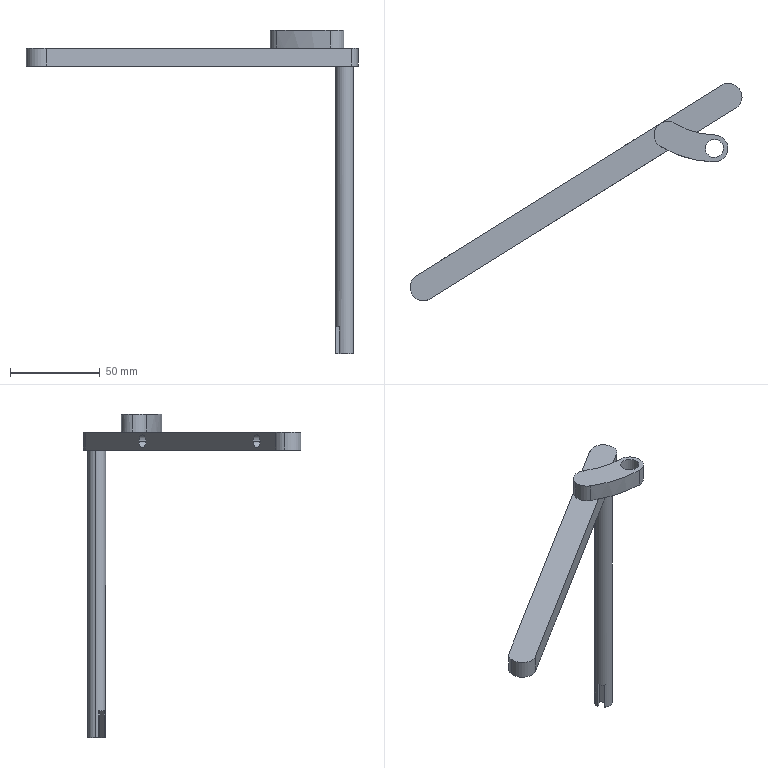Component | SolidWorks | DRocker(Left)-2 | 1 solid | 30 faces | box 184.66 x 120.91 x 180 mm | volume 48377 mm3 | cylinder 16 | plane 14 | commonest cylinder face diameters 15 x6 7 x4 10 x4 120 x1 90 x1
STEP:
#1=CARTESIAN_POINT('',(-10.505,0.6099,4.81));
#2=VERTEX_POINT('',#1);
#3=CARTESIAN_POINT('',(-10.738,0.464,4.81));
#4=VERTEX_POINT('',#3);
#5=CARTESIAN_POINT('',(-10.621,0.537,4.81));
#6=DIRECTION('',(-0.5295,0.8483,0.));
#7=DIRECTION('',(-0.8483,-0.5295,0.));
#8=AXIS2_PLACEMENT_3D('',#5,#6,#7);
#9=CIRCLE('',#8,0.1378);
#10=EDGE_CURVE('',#2,#4,#9,.T.);
#11=ORIENTED_EDGE('',*,*,#10,.F.);
#12=CARTESIAN_POINT('',(-10.713,0.9439,4.81));
#13=VERTEX_POINT('',#12);
#14=CARTESIAN_POINT('',(-10.505,0.6099,4.81));
#15=DIRECTION('',(-0.5295,0.8483,0.));
#16=VECTOR('',#15,39.37);
#17=LINE('',#14,#16);
#18=EDGE_CURVE('',#2,#13,#17,.T.);
#19=ORIENTED_EDGE('',*,*,#18,.T.);
#20=CARTESIAN_POINT('',(-10.947,0.798,4.81));
#21=VERTEX_POINT('',#20);
#22=CARTESIAN_POINT('',(-10.83,0.8709,4.81));
#23=DIRECTION('',(-0.5295,0.8483,0.));
#24=DIRECTION('',(-0.8483,-0.5295,0.));
#25=AXIS2_PLACEMENT_3D('',#22,#23,#24);
#26=CIRCLE('',#25,0.1378);
#27=EDGE_CURVE('',#13,#21,#26,.T.);
#28=ORIENTED_EDGE('',*,*,#27,.T.);
#29=CARTESIAN_POINT('',(-10.738,0.464,4.81));
#30=DIRECTION('',(-0.5295,0.8483,0.));
#31=VECTOR('',#30,39.37);
#32=LINE('',#29,#31);
#33=EDGE_CURVE('',#4,#21,#32,.T.);
#34=ORIENTED_EDGE('',*,*,#33,.F.);
#35=EDGE_LOOP('',(#11,#19,#28,#34));
#36=FACE_OUTER_BOUND('',#35,.T.);
#37=CARTESIAN_POINT('',(-10.621,0.537,4.81));
#38=DIRECTION('',(-0.5295,0.8483,0.));
#39=DIRECTION('',(-0.8483,-0.5295,0.));
#40=AXIS2_PLACEMENT_3D('',#37,#38,#39);
#41=CYLINDRICAL_SURFACE('',#40,0.1378);
#42=ADVANCED_FACE('',(#36),#41,.F.);
#43=CARTESIAN_POINT('',(-14.512,-1.892,4.81));
#44=VERTEX_POINT('',#43);
#45=CARTESIAN_POINT('',(-14.746,-2.038,4.81));
#46=VERTEX_POINT('',#45);
#47=CARTESIAN_POINT('',(-14.629,-1.965,4.81));
#48=DIRECTION('',(-0.5295,0.8483,0.));
#49=DIRECTION('',(-0.8483,-0.5295,0.));
#50=AXIS2_PLACEMENT_3D('',#47,#48,#49);
#51=CIRCLE('',#50,0.1378);
#52=EDGE_CURVE('',#44,#46,#51,.T.);
#53=ORIENTED_EDGE('',*,*,#52,.F.);
#54=CARTESIAN_POINT('',(-14.721,-1.558,4.81));
#55=VERTEX_POINT('',#54);
#56=CARTESIAN_POINT('',(-14.512,-1.892,4.81));
#57=DIRECTION('',(-0.5295,0.8483,0.));
#58=VECTOR('',#57,39.37);
#59=LINE('',#56,#58);
#60=EDGE_CURVE('',#44,#55,#59,.T.);
#61=ORIENTED_EDGE('',*,*,#60,.T.);
#62=CARTESIAN_POINT('',(-14.954,-1.704,4.81));
#63=VERTEX_POINT('',#62);
#64=CARTESIAN_POINT('',(-14.838,-1.631,4.81));
#65=DIRECTION('',(-0.5295,0.8483,0.));
#66=DIRECTION('',(-0.8483,-0.5295,0.));
#67=AXIS2_PLACEMENT_3D('',#64,#65,#66);
#68=CIRCLE('',#67,0.1378);
#69=EDGE_CURVE('',#55,#63,#68,.T.);
#70=ORIENTED_EDGE('',*,*,#69,.T.);
#71=CARTESIAN_POINT('',(-14.746,-2.038,4.81));
#72=DIRECTION('',(-0.5295,0.8483,0.));
#73=VECTOR('',#72,39.37);
#74=LINE('',#71,#73);
#75=EDGE_CURVE('',#46,#63,#74,.T.);
#76=ORIENTED_EDGE('',*,*,#75,.F.);
#77=EDGE_LOOP('',(#53,#61,#70,#76));
#78=FACE_OUTER_BOUND('',#77,.T.);
#79=CARTESIAN_POINT('',(-14.629,-1.965,4.81));
#80=DIRECTION('',(-0.5295,0.8483,0.));
#81=DIRECTION('',(-0.8483,-0.5295,0.));
#82=AXIS2_PLACEMENT_3D('',#79,#80,#81);
#83=CYLINDRICAL_SURFACE('',#82,0.1378);
#84=ADVANCED_FACE('',(#78),#83,.F.);
#85=CARTESIAN_POINT('',(-9.172,0.7751,5.401));
#86=VERTEX_POINT('',#85);
#87=CARTESIAN_POINT('',(-8.785,0.7031,5.401));
#88=VERTEX_POINT('',#87);
#89=CARTESIAN_POINT('',(-8.978,0.7391,5.401));
#90=DIRECTION('',(0.,0.,1.));
#91=DIRECTION('',(0.9831,-0.1829,0.));
#92=AXIS2_PLACEMENT_3D('',#89,#90,#91);
#93=CIRCLE('',#92,0.1969);
#94=EDGE_CURVE('',#86,#88,#93,.T.);
#95=ORIENTED_EDGE('',*,*,#94,.T.);
#96=CARTESIAN_POINT('',(-8.785,0.7031,5.007));
#97=VERTEX_POINT('',#96);
#98=CARTESIAN_POINT('',(-8.785,0.7031,5.401));
#99=DIRECTION('',(-0.,-0.,-1.));
#100=VECTOR('',#99,39.37);
#101=LINE('',#98,#100);
#102=EDGE_CURVE('',#88,#97,#101,.T.);
#103=ORIENTED_EDGE('',*,*,#102,.T.);
#104=CARTESIAN_POINT('',(-9.172,0.7751,5.007));
#105=VERTEX_POINT('',#104);
#106=CARTESIAN_POINT('',(-8.978,0.7391,5.007));
#107=DIRECTION('',(0.,0.,1.));
#108=DIRECTION('',(0.9831,-0.1829,0.));
#109=AXIS2_PLACEMENT_3D('',#106,#107,#108);
#110=CIRCLE('',#109,0.1969);
#111=EDGE_CURVE('',#105,#97,#110,.T.);
#112=ORIENTED_EDGE('',*,*,#111,.F.);
#113=CARTESIAN_POINT('',(-9.172,0.7751,5.401));
#114=DIRECTION('',(-0.,-0.,-1.));
#115=VECTOR('',#114,39.37);
#116=LINE('',#113,#115);
#117=EDGE_CURVE('',#86,#105,#116,.T.);
#118=ORIENTED_EDGE('',*,*,#117,.F.);
#119=EDGE_LOOP('',(#95,#103,#112,#118));
#120=FACE_OUTER_BOUND('',#119,.T.);
#121=CARTESIAN_POINT('',(-8.978,0.7391,5.401));
#122=DIRECTION('',(-0.,-0.,-1.));
#123=DIRECTION('',(-0.9831,0.1829,0.));
#124=AXIS2_PLACEMENT_3D('',#121,#122,#123);
#125=CYLINDRICAL_SURFACE('',#124,0.1969);
#126=ADVANCED_FACE('',(#120),#125,.F.);
#127=CARTESIAN_POINT('',(-10.296,1.091,5.401));
#128=VERTEX_POINT('',#127);
#129=CARTESIAN_POINT('',(-10.159,0.7848,5.401));
#130=VERTEX_POINT('',#129);
#131=CARTESIAN_POINT('',(-10.006,1.037,5.401));
#132=DIRECTION('',(0.,0.,1.));
#133=DIRECTION('',(0.9831,-0.1829,0.));
#134=AXIS2_PLACEMENT_3D('',#131,#132,#133);
#135=CIRCLE('',#134,0.2953);
#136=EDGE_CURVE('',#128,#130,#135,.T.);
#137=ORIENTED_EDGE('',*,*,#136,.F.);
#138=CARTESIAN_POINT('',(-10.296,1.091,5.007));
#139=VERTEX_POINT('',#138);
#140=CARTESIAN_POINT('',(-10.296,1.091,5.401));
#141=DIRECTION('',(-0.,-0.,-1.));
#142=VECTOR('',#141,39.37);
#143=LINE('',#140,#142);
#144=EDGE_CURVE('',#128,#139,#143,.T.);
#145=ORIENTED_EDGE('',*,*,#144,.T.);
#146=CARTESIAN_POINT('',(-10.159,0.7848,5.007));
#147=VERTEX_POINT('',#146);
#148=CARTESIAN_POINT('',(-10.006,1.037,5.007));
#149=DIRECTION('',(0.,0.,1.));
#150=DIRECTION('',(0.9831,-0.1829,0.));
#151=AXIS2_PLACEMENT_3D('',#148,#149,#150);
#152=CIRCLE('',#151,0.2953);
#153=EDGE_CURVE('',#139,#147,#152,.T.);
#154=ORIENTED_EDGE('',*,*,#153,.T.);
#155=CARTESIAN_POINT('',(-10.159,0.7848,5.401));
#156=DIRECTION('',(-0.,-0.,-1.));
#157=VECTOR('',#156,39.37);
#158=LINE('',#155,#157);
#159=EDGE_CURVE('',#130,#147,#158,.T.);
#160=ORIENTED_EDGE('',*,*,#159,.F.);
#161=EDGE_LOOP('',(#137,#145,#154,#160));
#162=FACE_OUTER_BOUND('',#161,.T.);
#163=CARTESIAN_POINT('',(-10.006,1.037,5.401));
#164=DIRECTION('',(-0.,-0.,-1.));
#165=DIRECTION('',(-0.9831,0.1829,0.));
#166=AXIS2_PLACEMENT_3D('',#163,#164,#165);
#167=CYLINDRICAL_SURFACE('',#166,0.2953);
#168=ADVANCED_FACE('',(#162),#167,.T.);
#169=CARTESIAN_POINT('',(-8.476,1.835,-1.686));
#170=VERTEX_POINT('',#169);
#171=CARTESIAN_POINT('',(-8.863,1.907,-1.686));
#172=VERTEX_POINT('',#171);
#173=CARTESIAN_POINT('',(-8.67,1.871,-1.686));
#174=DIRECTION('',(0.,0.,1.));
#175=DIRECTION('',(0.9831,-0.1829,0.));
#176=AXIS2_PLACEMENT_3D('',#173,#174,#175);
#177=CIRCLE('',#176,0.1969);
#178=EDGE_CURVE('',#170,#172,#177,.T.);
#179=ORIENTED_EDGE('',*,*,#178,.T.);
#180=CARTESIAN_POINT('',(-8.863,1.907,4.613));
#181=VERTEX_POINT('',#180);
#182=CARTESIAN_POINT('',(-8.863,1.907,-1.686));
#183=DIRECTION('',(0.,0.,1.));
#184=VECTOR('',#183,39.37);
#185=LINE('',#182,#184);
#186=EDGE_CURVE('',#172,#181,#185,.T.);
#187=ORIENTED_EDGE('',*,*,#186,.T.);
#188=CARTESIAN_POINT('',(-8.476,1.835,4.613));
#189=VERTEX_POINT('',#188);
#190=CARTESIAN_POINT('',(-8.67,1.871,4.613));
#191=DIRECTION('',(0.,0.,1.));
#192=DIRECTION('',(0.9831,-0.1829,0.));
#193=AXIS2_PLACEMENT_3D('',#190,#191,#192);
#194=CIRCLE('',#193,0.1969);
#195=EDGE_CURVE('',#189,#181,#194,.T.);
#196=ORIENTED_EDGE('',*,*,#195,.F.);
#197=CARTESIAN_POINT('',(-8.476,1.835,-1.686));
#198=DIRECTION('',(0.,0.,1.));
#199=VECTOR('',#198,39.37);
#200=LINE('',#197,#199);
#201=EDGE_CURVE('',#170,#189,#200,.T.);
#202=ORIENTED_EDGE('',*,*,#201,.F.);
#203=EDGE_LOOP('',(#179,#187,#196,#202));
#204=FACE_OUTER_BOUND('',#203,.T.);
#205=CARTESIAN_POINT('',(-8.67,1.871,-1.686));
#206=DIRECTION('',(0.,0.,1.));
#207=DIRECTION('',(0.9831,-0.1829,0.));
#208=AXIS2_PLACEMENT_3D('',#205,#206,#207);
#209=CYLINDRICAL_SURFACE('',#208,0.1969);
#210=ADVANCED_FACE('',(#204),#209,.T.);
#211=CARTESIAN_POINT('',(-15.639,-2.244,5.007));
#212=VERTEX_POINT('',#211);
#213=CARTESIAN_POINT('',(-15.193,-2.549,5.007));
#214=VERTEX_POINT('',#213);
#215=CARTESIAN_POINT('',(-15.349,-2.298,5.007));
#216=DIRECTION('',(0.,0.,1.));
#217=DIRECTION('',(0.9831,-0.1829,0.));
#218=AXIS2_PLACEMENT_3D('',#215,#216,#217);
#219=CIRCLE('',#218,0.2953);
#220=EDGE_CURVE('',#212,#214,#219,.T.);
#221=ORIENTED_EDGE('',*,*,#220,.F.);
#222=CARTESIAN_POINT('',(-15.639,-2.244,4.613));
#223=VERTEX_POINT('',#222);
#224=CARTESIAN_POINT('',(-15.639,-2.244,5.007));
#225=DIRECTION('',(-0.,-0.,-1.));
#226=VECTOR('',#225,39.37);
#227=LINE('',#224,#226);
#228=EDGE_CURVE('',#212,#223,#227,.T.);
#229=ORIENTED_EDGE('',*,*,#228,.T.);
#230=CARTESIAN_POINT('',(-15.193,-2.549,4.613));
#231=VERTEX_POINT('',#230);
#232=CARTESIAN_POINT('',(-15.349,-2.298,4.613));
#233=DIRECTION('',(0.,0.,1.));
#234=DIRECTION('',(0.9831,-0.1829,0.));
#235=AXIS2_PLACEMENT_3D('',#232,#233,#234);
#236=CIRCLE('',#235,0.2953);
#237=EDGE_CURVE('',#223,#231,#236,.T.);
#238=ORIENTED_EDGE('',*,*,#237,.T.);
#239=CARTESIAN_POINT('',(-15.193,-2.549,5.007));
#240=DIRECTION('',(-0.,-0.,-1.));
#241=VECTOR('',#240,39.37);
#242=LINE('',#239,#241);
#243=EDGE_CURVE('',#214,#231,#242,.T.);
#244=ORIENTED_EDGE('',*,*,#243,.F.);
#245=EDGE_LOOP('',(#221,#229,#238,#244));
#246=FACE_OUTER_BOUND('',#245,.T.);
#247=CARTESIAN_POINT('',(-15.349,-2.298,5.007));
#248=DIRECTION('',(-0.,-0.,-1.));
#249=DIRECTION('',(-0.9831,0.1829,0.));
#250=AXIS2_PLACEMENT_3D('',#247,#248,#249);
#251=CYLINDRICAL_SURFACE('',#250,0.2953);
#252=ADVANCED_FACE('',(#246),#251,.T.);
#253=CARTESIAN_POINT('',(-9.996,0.6951,5.007));
#254=VERTEX_POINT('',#253);
#255=CARTESIAN_POINT('',(-5.358,3.591,5.007));
#256=DIRECTION('',(-0.8483,-0.5295,0.));
#257=VECTOR('',#256,39.37);
#258=LINE('',#255,#257);
#259=EDGE_CURVE('',#254,#214,#258,.T.);
#260=ORIENTED_EDGE('',*,*,#259,.F.);
#261=CARTESIAN_POINT('',(-8.935,2.806,5.007));
#262=DIRECTION('',(0.,0.,1.));
#263=DIRECTION('',(0.9831,-0.1829,0.));
#264=AXIS2_PLACEMENT_3D('',#261,#262,#263);
#265=CIRCLE('',#264,2.362);
#266=EDGE_CURVE('',#147,#254,#265,.T.);
#267=ORIENTED_EDGE('',*,*,#266,.F.);
#268=ORIENTED_EDGE('',*,*,#153,.F.);
#269=CARTESIAN_POINT('',(-10.162,1.288,5.007));
#270=VERTEX_POINT('',#269);
#271=CARTESIAN_POINT('',(-10.006,1.037,5.007));
#272=DIRECTION('',(0.,0.,1.));
#273=DIRECTION('',(0.9831,-0.1829,0.));
#274=AXIS2_PLACEMENT_3D('',#271,#272,#273);
#275=CIRCLE('',#274,0.2953);
#276=EDGE_CURVE('',#270,#139,#275,.T.);
#277=ORIENTED_EDGE('',*,*,#276,.F.);
#278=CARTESIAN_POINT('',(-15.506,-2.048,5.007));
#279=VERTEX_POINT('',#278);
#280=CARTESIAN_POINT('',(-5.671,4.092,5.007));
#281=DIRECTION('',(-0.8483,-0.5295,0.));
#282=VECTOR('',#281,39.37);
#283=LINE('',#280,#282);
#284=EDGE_CURVE('',#270,#279,#283,.T.);
#285=ORIENTED_EDGE('',*,*,#284,.T.);
#286=CARTESIAN_POINT('',(-15.349,-2.298,5.007));
#287=DIRECTION('',(0.,0.,1.));
#288=DIRECTION('',(0.9831,-0.1829,0.));
#289=AXIS2_PLACEMENT_3D('',#286,#287,#288);
#290=CIRCLE('',#289,0.2953);
#291=EDGE_CURVE('',#279,#212,#290,.T.);
#292=ORIENTED_EDGE('',*,*,#291,.T.);
#293=ORIENTED_EDGE('',*,*,#220,.T.);
#294=EDGE_LOOP('',(#260,#267,#268,#277,#285,#292,#293));
#295=FACE_OUTER_BOUND('',#294,.T.);
#296=CARTESIAN_POINT('',(-1.007,-3.379,5.007));
#297=DIRECTION('',(0.,0.,1.));
#298=DIRECTION('',(0.9831,-0.1829,-0.));
#299=AXIS2_PLACEMENT_3D('',#296,#297,#298);
#300=PLANE('',#299);
#301=ADVANCED_FACE('',(#295),#300,.T.);
#302=CARTESIAN_POINT('',(-8.826,2.122,5.007));
#303=VERTEX_POINT('',#302);
#304=CARTESIAN_POINT('',(-5.671,4.092,5.007));
#305=DIRECTION('',(-0.8483,-0.5295,0.));
#306=VECTOR('',#305,39.37);
#307=LINE('',#304,#306);
#308=EDGE_CURVE('',#303,#270,#307,.T.);
#309=ORIENTED_EDGE('',*,*,#308,.T.);
#310=CARTESIAN_POINT('',(-9.853,1.29,5.007));
#311=VERTEX_POINT('',#310);
#312=CARTESIAN_POINT('',(-10.006,1.037,5.007));
#313=DIRECTION('',(0.,0.,1.));
#314=DIRECTION('',(0.9831,-0.1829,0.));
#315=AXIS2_PLACEMENT_3D('',#312,#313,#314);
#316=CIRCLE('',#315,0.2953);
#317=EDGE_CURVE('',#311,#270,#316,.T.);
#318=ORIENTED_EDGE('',*,*,#317,.F.);
#319=CARTESIAN_POINT('',(-9.368,1.088,5.007));
#320=VERTEX_POINT('',#319);
#321=CARTESIAN_POINT('',(-8.935,2.806,5.007));
#322=DIRECTION('',(-0.,-0.,-1.));
#323=DIRECTION('',(0.9831,-0.1829,0.));
#324=AXIS2_PLACEMENT_3D('',#321,#322,#323);
#325=CIRCLE('',#324,1.772);
#326=EDGE_CURVE('',#320,#311,#325,.T.);
#327=ORIENTED_EDGE('',*,*,#326,.F.);
#328=CARTESIAN_POINT('',(-8.513,1.621,5.007));
#329=VERTEX_POINT('',#328);
#330=CARTESIAN_POINT('',(-5.358,3.591,5.007));
#331=DIRECTION('',(-0.8483,-0.5295,0.));
#332=VECTOR('',#331,39.37);
#333=LINE('',#330,#332);
#334=EDGE_CURVE('',#329,#320,#333,.T.);
#335=ORIENTED_EDGE('',*,*,#334,.F.);
#336=CARTESIAN_POINT('',(-8.67,1.871,5.007));
#337=DIRECTION('',(0.,0.,1.));
#338=DIRECTION('',(0.9831,-0.1829,0.));
#339=AXIS2_PLACEMENT_3D('',#336,#337,#338);
#340=CIRCLE('',#339,0.2953);
#341=EDGE_CURVE('',#329,#303,#340,.T.);
#342=ORIENTED_EDGE('',*,*,#341,.T.);
#343=EDGE_LOOP('',(#309,#318,#327,#335,#342));
#344=FACE_OUTER_BOUND('',#343,.T.);
#345=CARTESIAN_POINT('',(-1.007,-3.379,5.007));
#346=DIRECTION('',(0.,0.,1.));
#347=DIRECTION('',(0.9831,-0.1829,-0.));
#348=AXIS2_PLACEMENT_3D('',#345,#346,#347);
#349=PLANE('',#348);
#350=ADVANCED_FACE('',(#344),#349,.T.);
#351=CARTESIAN_POINT('',(-10.83,0.8709,4.81));
#352=DIRECTION('',(-0.5295,0.8483,0.));
#353=DIRECTION('',(-0.8483,-0.5295,0.));
#354=AXIS2_PLACEMENT_3D('',#351,#352,#353);
#355=CIRCLE('',#354,0.1378);
#356=EDGE_CURVE('',#21,#13,#355,.T.);
#357=ORIENTED_EDGE('',*,*,#356,.F.);
#358=ORIENTED_EDGE('',*,*,#27,.F.);
#359=EDGE_LOOP('',(#357,#358));
#360=FACE_BOUND('',#359,.T.);
#361=CARTESIAN_POINT('',(-14.838,-1.631,4.81));
#362=DIRECTION('',(-0.5295,0.8483,0.));
#363=DIRECTION('',(-0.8483,-0.5295,0.));
#364=AXIS2_PLACEMENT_3D('',#361,#362,#363);
#365=CIRCLE('',#364,0.1378);
#366=EDGE_CURVE('',#63,#55,#365,.T.);
#367=ORIENTED_EDGE('',*,*,#366,.F.);
#368=ORIENTED_EDGE('',*,*,#69,.F.);
#369=EDGE_LOOP('',(#367,#368));
#370=FACE_BOUND('',#369,.T.);
#371=CARTESIAN_POINT('',(-8.826,2.122,4.613));
#372=VERTEX_POINT('',#371);
#373=CARTESIAN_POINT('',(-15.506,-2.048,4.613));
#374=VERTEX_POINT('',#373);
#375=CARTESIAN_POINT('',(-5.671,4.092,4.613));
#376=DIRECTION('',(-0.8483,-0.5295,0.));
#377=VECTOR('',#376,39.37);
#378=LINE('',#375,#377);
#379=EDGE_CURVE('',#372,#374,#378,.T.);
#380=ORIENTED_EDGE('',*,*,#379,.T.);
#381=CARTESIAN_POINT('',(-15.506,-2.048,5.007));
#382=DIRECTION('',(-0.,-0.,-1.));
#383=VECTOR('',#382,39.37);
#384=LINE('',#381,#383);
#385=EDGE_CURVE('',#279,#374,#384,.T.);
#386=ORIENTED_EDGE('',*,*,#385,.F.);
#387=ORIENTED_EDGE('',*,*,#284,.F.);
#388=ORIENTED_EDGE('',*,*,#308,.F.);
#389=CARTESIAN_POINT('',(-8.826,2.122,5.007));
#390=DIRECTION('',(-0.,-0.,-1.));
#391=VECTOR('',#390,39.37);
#392=LINE('',#389,#391);
#393=EDGE_CURVE('',#303,#372,#392,.T.);
#394=ORIENTED_EDGE('',*,*,#393,.T.);
#395=EDGE_LOOP('',(#380,#386,#387,#388,#394));
#396=FACE_OUTER_BOUND('',#395,.T.);
#397=CARTESIAN_POINT('',(-5.671,4.092,5.007));
#398=DIRECTION('',(0.5295,-0.8483,-0.));
#399=DIRECTION('',(0.8483,0.5295,-0.));
#400=AXIS2_PLACEMENT_3D('',#397,#398,#399);
#401=PLANE('',#400);
#402=ADVANCED_FACE('',(#360,#370,#396),#401,.F.);
#403=ORIENTED_EDGE('',*,*,#228,.F.);
#404=ORIENTED_EDGE('',*,*,#291,.F.);
#405=ORIENTED_EDGE('',*,*,#385,.T.);
#406=CARTESIAN_POINT('',(-15.349,-2.298,4.613));
#407=DIRECTION('',(0.,0.,1.));
#408=DIRECTION('',(0.9831,-0.1829,0.));
#409=AXIS2_PLACEMENT_3D('',#406,#407,#408);
#410=CIRCLE('',#409,0.2953);
#411=EDGE_CURVE('',#374,#223,#410,.T.);
#412=ORIENTED_EDGE('',*,*,#411,.T.);
#413=EDGE_LOOP('',(#403,#404,#405,#412));
#414=FACE_OUTER_BOUND('',#413,.T.);
#415=CARTESIAN_POINT('',(-15.349,-2.298,5.007));
#416=DIRECTION('',(-0.,-0.,-1.));
#417=DIRECTION('',(-0.9831,0.1829,0.));
#418=AXIS2_PLACEMENT_3D('',#415,#416,#417);
#419=CYLINDRICAL_SURFACE('',#418,0.2953);
#420=ADVANCED_FACE('',(#414),#419,.T.);
#421=CARTESIAN_POINT('',(-8.513,1.621,4.613));
#422=VERTEX_POINT('',#421);
#423=CARTESIAN_POINT('',(-5.358,3.591,4.613));
#424=DIRECTION('',(-0.8483,-0.5295,0.));
#425=VECTOR('',#424,39.37);
#426=LINE('',#423,#425);
#427=EDGE_CURVE('',#422,#231,#426,.T.);
#428=ORIENTED_EDGE('',*,*,#427,.F.);
#429=CARTESIAN_POINT('',(-8.513,1.621,5.007));
#430=DIRECTION('',(-0.,-0.,-1.));
#431=VECTOR('',#430,39.37);
#432=LINE('',#429,#431);
#433=EDGE_CURVE('',#329,#422,#432,.T.);
#434=ORIENTED_EDGE('',*,*,#433,.F.);
#435=ORIENTED_EDGE('',*,*,#334,.T.);
#436=CARTESIAN_POINT('',(-5.358,3.591,5.007));
#437=DIRECTION('',(-0.8483,-0.5295,0.));
#438=VECTOR('',#437,39.37);
#439=LINE('',#436,#438);
#440=EDGE_CURVE('',#320,#254,#439,.T.);
#441=ORIENTED_EDGE('',*,*,#440,.T.);
#442=ORIENTED_EDGE('',*,*,#259,.T.);
#443=ORIENTED_EDGE('',*,*,#243,.T.);
#444=EDGE_LOOP('',(#428,#434,#435,#441,#442,#443));
#445=FACE_OUTER_BOUND('',#444,.T.);
#446=CARTESIAN_POINT('',(-5.358,3.591,5.007));
#447=DIRECTION('',(0.5295,-0.8483,-0.));
#448=DIRECTION('',(0.8483,0.5295,-0.));
#449=AXIS2_PLACEMENT_3D('',#446,#447,#448);
#450=PLANE('',#449);
#451=ADVANCED_FACE('',(#445),#450,.T.);
#452=CARTESIAN_POINT('',(-8.67,1.871,4.613));
#453=DIRECTION('',(0.,0.,1.));
#454=DIRECTION('',(0.9831,-0.1829,0.));
#455=AXIS2_PLACEMENT_3D('',#452,#453,#454);
#456=CIRCLE('',#455,0.2953);
#457=EDGE_CURVE('',#422,#372,#456,.T.);
#458=ORIENTED_EDGE('',*,*,#457,.T.);
#459=ORIENTED_EDGE('',*,*,#393,.F.);
#460=ORIENTED_EDGE('',*,*,#341,.F.);
#461=ORIENTED_EDGE('',*,*,#433,.T.);
#462=EDGE_LOOP('',(#458,#459,#460,#461));
#463=FACE_OUTER_BOUND('',#462,.T.);
#464=CARTESIAN_POINT('',(-8.67,1.871,5.007));
#465=DIRECTION('',(-0.,-0.,-1.));
#466=DIRECTION('',(-0.9831,0.1829,0.));
#467=AXIS2_PLACEMENT_3D('',#464,#465,#466);
#468=CYLINDRICAL_SURFACE('',#467,0.2953);
#469=ADVANCED_FACE('',(#463),#468,.T.);
#470=ORIENTED_EDGE('',*,*,#195,.T.);
#471=CARTESIAN_POINT('',(-8.67,1.871,4.613));
#472=DIRECTION('',(0.,0.,1.));
#473=DIRECTION('',(0.9831,-0.1829,0.));
#474=AXIS2_PLACEMENT_3D('',#471,#472,#473);
#475=CIRCLE('',#474,0.1969);
#476=EDGE_CURVE('',#181,#189,#475,.T.);
#477=ORIENTED_EDGE('',*,*,#476,.T.);
#478=EDGE_LOOP('',(#470,#477));
#479=FACE_BOUND('',#478,.T.);
#480=ORIENTED_EDGE('',*,*,#379,.F.);
#481=ORIENTED_EDGE('',*,*,#457,.F.);
#482=ORIENTED_EDGE('',*,*,#427,.T.);
#483=ORIENTED_EDGE('',*,*,#237,.F.);
#484=ORIENTED_EDGE('',*,*,#411,.F.);
#485=EDGE_LOOP('',(#480,#481,#482,#483,#484));
#486=FACE_OUTER_BOUND('',#485,.T.);
#487=CARTESIAN_POINT('',(-1.007,-3.379,4.613));
#488=DIRECTION('',(0.,0.,1.));
#489=DIRECTION('',(0.9831,-0.1829,-0.));
#490=AXIS2_PLACEMENT_3D('',#487,#488,#489);
#491=PLANE('',#490);
#492=ADVANCED_FACE('',(#479,#486),#491,.F.);
#493=ORIENTED_EDGE('',*,*,#186,.F.);
#494=CARTESIAN_POINT('',(-8.864,1.843,-1.686));
#495=VERTEX_POINT('',#494);
#496=CARTESIAN_POINT('',(-8.67,1.871,-1.686));
#497=DIRECTION('',(0.,0.,1.));
#498=DIRECTION('',(0.9831,-0.1829,0.));
#499=AXIS2_PLACEMENT_3D('',#496,#497,#498);
#500=CIRCLE('',#499,0.1969);
#501=EDGE_CURVE('',#172,#495,#500,.T.);
#502=ORIENTED_EDGE('',*,*,#501,.T.);
#503=CARTESIAN_POINT('',(-8.864,1.843,-1.095));
#504=VERTEX_POINT('',#503);
#505=CARTESIAN_POINT('',(-8.864,1.843,-1.686));
#506=DIRECTION('',(-0.,-0.,-1.));
#507=VECTOR('',#506,39.37);
#508=LINE('',#505,#507);
#509=EDGE_CURVE('',#504,#495,#508,.T.);
#510=ORIENTED_EDGE('',*,*,#509,.F.);
#511=CARTESIAN_POINT('',(-8.781,1.709,-1.095));
#512=VERTEX_POINT('',#511);
#513=CARTESIAN_POINT('',(-8.67,1.871,-1.095));
#514=DIRECTION('',(0.,0.,1.));
#515=DIRECTION('',(-0.9831,0.1829,0.));
#516=AXIS2_PLACEMENT_3D('',#513,#514,#515);
#517=CIRCLE('',#516,0.1969);
#518=EDGE_CURVE('',#504,#512,#517,.T.);
#519=ORIENTED_EDGE('',*,*,#518,.T.);
#520=CARTESIAN_POINT('',(-8.781,1.709,-1.686));
#521=VERTEX_POINT('',#520);
#522=CARTESIAN_POINT('',(-8.781,1.709,-1.686));
#523=DIRECTION('',(0.,0.,1.));
#524=VECTOR('',#523,39.37);
#525=LINE('',#522,#524);
#526=EDGE_CURVE('',#521,#512,#525,.T.);
#527=ORIENTED_EDGE('',*,*,#526,.F.);
#528=CARTESIAN_POINT('',(-8.67,1.871,-1.686));
#529=DIRECTION('',(0.,0.,1.));
#530=DIRECTION('',(0.9831,-0.1829,0.));
#531=AXIS2_PLACEMENT_3D('',#528,#529,#530);
#532=CIRCLE('',#531,0.1969);
#533=EDGE_CURVE('',#521,#170,#532,.T.);
#534=ORIENTED_EDGE('',*,*,#533,.T.);
#535=ORIENTED_EDGE('',*,*,#201,.T.);
#536=ORIENTED_EDGE('',*,*,#476,.F.);
#537=EDGE_LOOP('',(#493,#502,#510,#519,#527,#534,#535,#536));
#538=FACE_OUTER_BOUND('',#537,.T.);
#539=CARTESIAN_POINT('',(-8.67,1.871,-1.686));
#540=DIRECTION('',(0.,0.,1.));
#541=DIRECTION('',(0.9831,-0.1829,0.));
#542=AXIS2_PLACEMENT_3D('',#539,#540,#541);
#543=CYLINDRICAL_SURFACE('',#542,0.1969);
#544=ADVANCED_FACE('',(#538),#543,.T.);
#545=ORIENTED_EDGE('',*,*,#533,.F.);
#546=CARTESIAN_POINT('',(-8.628,1.805,-1.686));
#547=VERTEX_POINT('',#546);
#548=CARTESIAN_POINT('',(-8.962,1.596,-1.686));
#549=DIRECTION('',(-0.8483,-0.5295,0.));
#550=VECTOR('',#549,39.37);
#551=LINE('',#548,#550);
#552=EDGE_CURVE('',#547,#521,#551,.T.);
#553=ORIENTED_EDGE('',*,*,#552,.F.);
#554=CARTESIAN_POINT('',(-8.711,1.938,-1.686));
#555=VERTEX_POINT('',#554);
#556=CARTESIAN_POINT('',(-8.628,1.805,-1.686));
#557=DIRECTION('',(0.5295,-0.8483,-0.));
#558=VECTOR('',#557,39.37);
#559=LINE('',#556,#558);
#560=EDGE_CURVE('',#555,#547,#559,.T.);
#561=ORIENTED_EDGE('',*,*,#560,.F.);
#562=CARTESIAN_POINT('',(-5.556,3.908,-1.686));
#563=DIRECTION('',(-0.8483,-0.5295,0.));
#564=VECTOR('',#563,39.37);
#565=LINE('',#562,#564);
#566=EDGE_CURVE('',#555,#495,#565,.T.);
#567=ORIENTED_EDGE('',*,*,#566,.T.);
#568=ORIENTED_EDGE('',*,*,#501,.F.);
#569=ORIENTED_EDGE('',*,*,#178,.F.);
#570=EDGE_LOOP('',(#545,#553,#561,#567,#568,#569));
#571=FACE_OUTER_BOUND('',#570,.T.);
#572=CARTESIAN_POINT('',(-1.007,-3.379,-1.686));
#573=DIRECTION('',(0.,0.,1.));
#574=DIRECTION('',(0.9831,-0.1829,-0.));
#575=AXIS2_PLACEMENT_3D('',#572,#573,#574);
#576=PLANE('',#575);
#577=ADVANCED_FACE('',(#571),#576,.F.);
#578=ORIENTED_EDGE('',*,*,#111,.T.);
#579=CARTESIAN_POINT('',(-8.978,0.7391,5.007));
#580=DIRECTION('',(0.,0.,1.));
#581=DIRECTION('',(0.9831,-0.1829,0.));
#582=AXIS2_PLACEMENT_3D('',#579,#580,#581);
#583=CIRCLE('',#582,0.1969);
#584=EDGE_CURVE('',#97,#105,#583,.T.);
#585=ORIENTED_EDGE('',*,*,#584,.T.);
#586=EDGE_LOOP('',(#578,#585));
#587=FACE_BOUND('',#586,.T.);
#588=ORIENTED_EDGE('',*,*,#440,.F.);
#589=CARTESIAN_POINT('',(-8.972,1.034,5.007));
#590=VERTEX_POINT('',#589);
#591=CARTESIAN_POINT('',(-8.935,2.806,5.007));
#592=DIRECTION('',(-0.,-0.,-1.));
#593=DIRECTION('',(0.9831,-0.1829,0.));
#594=AXIS2_PLACEMENT_3D('',#591,#592,#593);
#595=CIRCLE('',#594,1.772);
#596=EDGE_CURVE('',#590,#320,#595,.T.);
#597=ORIENTED_EDGE('',*,*,#596,.F.);
#598=CARTESIAN_POINT('',(-8.984,0.4439,5.007));
#599=VERTEX_POINT('',#598);
#600=CARTESIAN_POINT('',(-8.978,0.7391,5.007));
#601=DIRECTION('',(0.,0.,1.));
#602=DIRECTION('',(0.9831,-0.1829,0.));
#603=AXIS2_PLACEMENT_3D('',#600,#601,#602);
#604=CIRCLE('',#603,0.2953);
#605=EDGE_CURVE('',#599,#590,#604,.T.);
#606=ORIENTED_EDGE('',*,*,#605,.F.);
#607=CARTESIAN_POINT('',(-8.935,2.806,5.007));
#608=DIRECTION('',(0.,0.,1.));
#609=DIRECTION('',(0.9831,-0.1829,0.));
#610=AXIS2_PLACEMENT_3D('',#607,#608,#609);
#611=CIRCLE('',#610,2.362);
#612=EDGE_CURVE('',#254,#599,#611,.T.);
#613=ORIENTED_EDGE('',*,*,#612,.F.);
#614=EDGE_LOOP('',(#588,#597,#606,#613));
#615=FACE_OUTER_BOUND('',#614,.T.);
#616=CARTESIAN_POINT('',(-9.47,1.921,5.007));
#617=DIRECTION('',(0.,0.,1.));
#618=DIRECTION('',(0.9831,-0.1829,-0.));
#619=AXIS2_PLACEMENT_3D('',#616,#617,#618);
#620=PLANE('',#619);
#621=ADVANCED_FACE('',(#587,#615),#620,.F.);
#622=ORIENTED_EDGE('',*,*,#144,.F.);
#623=CARTESIAN_POINT('',(-9.853,1.29,5.401));
#624=VERTEX_POINT('',#623);
#625=CARTESIAN_POINT('',(-10.006,1.037,5.401));
#626=DIRECTION('',(0.,0.,1.));
#627=DIRECTION('',(0.9831,-0.1829,0.));
#628=AXIS2_PLACEMENT_3D('',#625,#626,#627);
#629=CIRCLE('',#628,0.2953);
#630=EDGE_CURVE('',#624,#128,#629,.T.);
#631=ORIENTED_EDGE('',*,*,#630,.F.);
#632=CARTESIAN_POINT('',(-9.853,1.29,5.401));
#633=DIRECTION('',(-0.,-0.,-1.));
#634=VECTOR('',#633,39.37);
#635=LINE('',#632,#634);
#636=EDGE_CURVE('',#624,#311,#635,.T.);
#637=ORIENTED_EDGE('',*,*,#636,.T.);
#638=ORIENTED_EDGE('',*,*,#317,.T.);
#639=ORIENTED_EDGE('',*,*,#276,.T.);
#640=EDGE_LOOP('',(#622,#631,#637,#638,#639));
#641=FACE_OUTER_BOUND('',#640,.T.);
#642=CARTESIAN_POINT('',(-10.006,1.037,5.401));
#643=DIRECTION('',(-0.,-0.,-1.));
#644=DIRECTION('',(-0.9831,0.1829,0.));
#645=AXIS2_PLACEMENT_3D('',#642,#643,#644);
#646=CYLINDRICAL_SURFACE('',#645,0.2953);
#647=ADVANCED_FACE('',(#641),#646,.T.);
#648=ORIENTED_EDGE('',*,*,#266,.T.);
#649=ORIENTED_EDGE('',*,*,#612,.T.);
#650=CARTESIAN_POINT('',(-8.984,0.4439,5.401));
#651=VERTEX_POINT('',#650);
#652=CARTESIAN_POINT('',(-8.984,0.4439,5.401));
#653=DIRECTION('',(-0.,-0.,-1.));
#654=VECTOR('',#653,39.37);
#655=LINE('',#652,#654);
#656=EDGE_CURVE('',#651,#599,#655,.T.);
#657=ORIENTED_EDGE('',*,*,#656,.F.);
#658=CARTESIAN_POINT('',(-8.935,2.806,5.401));
#659=DIRECTION('',(0.,0.,1.));
#660=DIRECTION('',(0.9831,-0.1829,0.));
#661=AXIS2_PLACEMENT_3D('',#658,#659,#660);
#662=CIRCLE('',#661,2.362);
#663=EDGE_CURVE('',#130,#651,#662,.T.);
#664=ORIENTED_EDGE('',*,*,#663,.F.);
#665=ORIENTED_EDGE('',*,*,#159,.T.);
#666=EDGE_LOOP('',(#648,#649,#657,#664,#665));
#667=FACE_OUTER_BOUND('',#666,.T.);
#668=CARTESIAN_POINT('',(-8.935,2.806,5.401));
#669=DIRECTION('',(-0.,-0.,-1.));
#670=DIRECTION('',(-0.9831,0.1829,0.));
#671=AXIS2_PLACEMENT_3D('',#668,#669,#670);
#672=CYLINDRICAL_SURFACE('',#671,2.362);
#673=ADVANCED_FACE('',(#667),#672,.T.);
#674=ORIENTED_EDGE('',*,*,#605,.T.);
#675=CARTESIAN_POINT('',(-8.972,1.034,5.401));
#676=VERTEX_POINT('',#675);
#677=CARTESIAN_POINT('',(-8.972,1.034,5.401));
#678=DIRECTION('',(-0.,-0.,-1.));
#679=VECTOR('',#678,39.37);
#680=LINE('',#677,#679);
#681=EDGE_CURVE('',#676,#590,#680,.T.);
#682=ORIENTED_EDGE('',*,*,#681,.F.);
#683=CARTESIAN_POINT('',(-8.978,0.7391,5.401));
#684=DIRECTION('',(0.,0.,1.));
#685=DIRECTION('',(0.9831,-0.1829,0.));
#686=AXIS2_PLACEMENT_3D('',#683,#684,#685);
#687=CIRCLE('',#686,0.2953);
#688=EDGE_CURVE('',#651,#676,#687,.T.);
#689=ORIENTED_EDGE('',*,*,#688,.F.);
#690=ORIENTED_EDGE('',*,*,#656,.T.);
#691=EDGE_LOOP('',(#674,#682,#689,#690));
#692=FACE_OUTER_BOUND('',#691,.T.);
#693=CARTESIAN_POINT('',(-8.978,0.7391,5.401));
#694=DIRECTION('',(-0.,-0.,-1.));
#695=DIRECTION('',(-0.9831,0.1829,0.));
#696=AXIS2_PLACEMENT_3D('',#693,#694,#695);
#697=CYLINDRICAL_SURFACE('',#696,0.2953);
#698=ADVANCED_FACE('',(#692),#697,.T.);
#699=ORIENTED_EDGE('',*,*,#596,.T.);
#700=ORIENTED_EDGE('',*,*,#326,.T.);
#701=ORIENTED_EDGE('',*,*,#636,.F.);
#702=CARTESIAN_POINT('',(-8.935,2.806,5.401));
#703=DIRECTION('',(-0.,-0.,-1.));
#704=DIRECTION('',(0.9831,-0.1829,0.));
#705=AXIS2_PLACEMENT_3D('',#702,#703,#704);
#706=CIRCLE('',#705,1.772);
#707=EDGE_CURVE('',#676,#624,#706,.T.);
#708=ORIENTED_EDGE('',*,*,#707,.F.);
#709=ORIENTED_EDGE('',*,*,#681,.T.);
#710=EDGE_LOOP('',(#699,#700,#701,#708,#709));
#711=FACE_OUTER_BOUND('',#710,.T.);
#712=CARTESIAN_POINT('',(-8.935,2.806,5.401));
#713=DIRECTION('',(-0.,-0.,-1.));
#714=DIRECTION('',(-0.9831,0.1829,0.));
#715=AXIS2_PLACEMENT_3D('',#712,#713,#714);
#716=CYLINDRICAL_SURFACE('',#715,1.772);
#717=ADVANCED_FACE('',(#711),#716,.F.);
#718=ORIENTED_EDGE('',*,*,#102,.F.);
#719=CARTESIAN_POINT('',(-8.978,0.7391,5.401));
#720=DIRECTION('',(0.,0.,1.));
#721=DIRECTION('',(0.9831,-0.1829,0.));
#722=AXIS2_PLACEMENT_3D('',#719,#720,#721);
#723=CIRCLE('',#722,0.1969);
#724=EDGE_CURVE('',#88,#86,#723,.T.);
#725=ORIENTED_EDGE('',*,*,#724,.T.);
#726=ORIENTED_EDGE('',*,*,#117,.T.);
#727=ORIENTED_EDGE('',*,*,#584,.F.);
#728=EDGE_LOOP('',(#718,#725,#726,#727));
#729=FACE_OUTER_BOUND('',#728,.T.);
#730=CARTESIAN_POINT('',(-8.978,0.7391,5.401));
#731=DIRECTION('',(-0.,-0.,-1.));
#732=DIRECTION('',(-0.9831,0.1829,0.));
#733=AXIS2_PLACEMENT_3D('',#730,#731,#732);
#734=CYLINDRICAL_SURFACE('',#733,0.1969);
#735=ADVANCED_FACE('',(#729),#734,.F.);
#736=ORIENTED_EDGE('',*,*,#630,.T.);
#737=ORIENTED_EDGE('',*,*,#136,.T.);
#738=ORIENTED_EDGE('',*,*,#663,.T.);
#739=ORIENTED_EDGE('',*,*,#688,.T.);
#740=ORIENTED_EDGE('',*,*,#707,.T.);
#741=EDGE_LOOP('',(#736,#737,#738,#739,#740));
#742=FACE_OUTER_BOUND('',#741,.T.);
#743=ORIENTED_EDGE('',*,*,#94,.F.);
#744=ORIENTED_EDGE('',*,*,#724,.F.);
#745=EDGE_LOOP('',(#743,#744));
#746=FACE_BOUND('',#745,.T.);
#747=CARTESIAN_POINT('',(-10.006,1.037,5.401));
#748=DIRECTION('',(0.,0.,1.));
#749=DIRECTION('',(0.9831,-0.1829,-0.));
#750=AXIS2_PLACEMENT_3D('',#747,#748,#749);
#751=PLANE('',#750);
#752=ADVANCED_FACE('',(#742,#746),#751,.T.);
#753=ORIENTED_EDGE('',*,*,#526,.T.);
#754=CARTESIAN_POINT('',(-8.628,1.805,-1.095));
#755=VERTEX_POINT('',#754);
#756=CARTESIAN_POINT('',(-8.962,1.596,-1.095));
#757=DIRECTION('',(-0.8483,-0.5295,0.));
#758=VECTOR('',#757,39.37);
#759=LINE('',#756,#758);
#760=EDGE_CURVE('',#755,#512,#759,.T.);
#761=ORIENTED_EDGE('',*,*,#760,.F.);
#762=CARTESIAN_POINT('',(-8.628,1.805,-1.095));
#763=DIRECTION('',(-0.,-0.,-1.));
#764=VECTOR('',#763,39.37);
#765=LINE('',#762,#764);
#766=EDGE_CURVE('',#755,#547,#765,.T.);
#767=ORIENTED_EDGE('',*,*,#766,.T.);
#768=ORIENTED_EDGE('',*,*,#552,.T.);
#769=EDGE_LOOP('',(#753,#761,#767,#768));
#770=FACE_OUTER_BOUND('',#769,.T.);
#771=CARTESIAN_POINT('',(-8.962,1.596,-1.095));
#772=DIRECTION('',(0.5295,-0.8483,-0.));
#773=DIRECTION('',(0.8483,0.5295,-0.));
#774=AXIS2_PLACEMENT_3D('',#771,#772,#773);
#775=PLANE('',#774);
#776=ADVANCED_FACE('',(#770),#775,.F.);
#777=ORIENTED_EDGE('',*,*,#560,.T.);
#778=ORIENTED_EDGE('',*,*,#766,.F.);
#779=CARTESIAN_POINT('',(-8.711,1.938,-1.095));
#780=VERTEX_POINT('',#779);
#781=CARTESIAN_POINT('',(-8.628,1.805,-1.095));
#782=DIRECTION('',(0.5295,-0.8483,-0.));
#783=VECTOR('',#782,39.37);
#784=LINE('',#781,#783);
#785=EDGE_CURVE('',#780,#755,#784,.T.);
#786=ORIENTED_EDGE('',*,*,#785,.F.);
#787=CARTESIAN_POINT('',(-8.711,1.938,-1.095));
#788=DIRECTION('',(-0.,-0.,-1.));
#789=VECTOR('',#788,39.37);
#790=LINE('',#787,#789);
#791=EDGE_CURVE('',#780,#555,#790,.T.);
#792=ORIENTED_EDGE('',*,*,#791,.T.);
#793=EDGE_LOOP('',(#777,#778,#786,#792));
#794=FACE_OUTER_BOUND('',#793,.T.);
#795=CARTESIAN_POINT('',(-8.628,1.805,-1.095));
#796=DIRECTION('',(0.8483,0.5295,-0.));
#797=DIRECTION('',(-0.5295,0.8483,0.));
#798=AXIS2_PLACEMENT_3D('',#795,#796,#797);
#799=PLANE('',#798);
#800=ADVANCED_FACE('',(#794),#799,.F.);
#801=ORIENTED_EDGE('',*,*,#509,.T.);
#802=ORIENTED_EDGE('',*,*,#566,.F.);
#803=ORIENTED_EDGE('',*,*,#791,.F.);
#804=CARTESIAN_POINT('',(-9.045,1.73,-1.095));
#805=DIRECTION('',(0.8483,0.5295,-0.));
#806=VECTOR('',#805,39.37);
#807=LINE('',#804,#806);
#808=EDGE_CURVE('',#504,#780,#807,.T.);
#809=ORIENTED_EDGE('',*,*,#808,.F.);
#810=EDGE_LOOP('',(#801,#802,#803,#809));
#811=FACE_OUTER_BOUND('',#810,.T.);
#812=CARTESIAN_POINT('',(-9.045,1.73,-1.095));
#813=DIRECTION('',(-0.5295,0.8483,0.));
#814=DIRECTION('',(-0.8483,-0.5295,0.));
#815=AXIS2_PLACEMENT_3D('',#812,#813,#814);
#816=PLANE('',#815);
#817=ADVANCED_FACE('',(#811),#816,.F.);
#818=ORIENTED_EDGE('',*,*,#808,.T.);
#819=ORIENTED_EDGE('',*,*,#785,.T.);
#820=ORIENTED_EDGE('',*,*,#760,.T.);
#821=ORIENTED_EDGE('',*,*,#518,.F.);
#822=EDGE_LOOP('',(#818,#819,#820,#821));
#823=FACE_OUTER_BOUND('',#822,.T.);
#824=CARTESIAN_POINT('',(-1.007,-3.379,-1.095));
#825=DIRECTION('',(-0.,-0.,-1.));
#826=DIRECTION('',(-0.9831,0.1829,0.));
#827=AXIS2_PLACEMENT_3D('',#824,#825,#826);
#828=PLANE('',#827);
#829=ADVANCED_FACE('',(#823),#828,.T.);
#830=ORIENTED_EDGE('',*,*,#60,.F.);
#831=CARTESIAN_POINT('',(-14.629,-1.965,4.81));
#832=DIRECTION('',(-0.5295,0.8483,0.));
#833=DIRECTION('',(-0.8483,-0.5295,0.));
#834=AXIS2_PLACEMENT_3D('',#831,#832,#833);
#835=CIRCLE('',#834,0.1378);
#836=EDGE_CURVE('',#46,#44,#835,.T.);
#837=ORIENTED_EDGE('',*,*,#836,.F.);
#838=ORIENTED_EDGE('',*,*,#75,.T.);
#839=ORIENTED_EDGE('',*,*,#366,.T.);
#840=EDGE_LOOP('',(#830,#837,#838,#839));
#841=FACE_OUTER_BOUND('',#840,.T.);
#842=CARTESIAN_POINT('',(-14.629,-1.965,4.81));
#843=DIRECTION('',(-0.5295,0.8483,0.));
#844=DIRECTION('',(-0.8483,-0.5295,0.));
#845=AXIS2_PLACEMENT_3D('',#842,#843,#844);
#846=CYLINDRICAL_SURFACE('',#845,0.1378);
#847=ADVANCED_FACE('',(#841),#846,.F.);
#848=ORIENTED_EDGE('',*,*,#836,.T.);
#849=ORIENTED_EDGE('',*,*,#52,.T.);
#850=EDGE_LOOP('',(#848,#849));
#851=FACE_OUTER_BOUND('',#850,.T.);
#852=CARTESIAN_POINT('',(-14.629,-1.965,4.81));
#853=DIRECTION('',(-0.5295,0.8483,0.));
#854=DIRECTION('',(-0.8483,-0.5295,0.));
#855=AXIS2_PLACEMENT_3D('',#852,#853,#854);
#856=PLANE('',#855);
#857=ADVANCED_FACE('',(#851),#856,.T.);
#858=ORIENTED_EDGE('',*,*,#18,.F.);
#859=CARTESIAN_POINT('',(-10.621,0.537,4.81));
#860=DIRECTION('',(-0.5295,0.8483,0.));
#861=DIRECTION('',(-0.8483,-0.5295,0.));
#862=AXIS2_PLACEMENT_3D('',#859,#860,#861);
#863=CIRCLE('',#862,0.1378);
#864=EDGE_CURVE('',#4,#2,#863,.T.);
#865=ORIENTED_EDGE('',*,*,#864,.F.);
#866=ORIENTED_EDGE('',*,*,#33,.T.);
#867=ORIENTED_EDGE('',*,*,#356,.T.);
#868=EDGE_LOOP('',(#858,#865,#866,#867));
#869=FACE_OUTER_BOUND('',#868,.T.);
#870=CARTESIAN_POINT('',(-10.621,0.537,4.81));
#871=DIRECTION('',(-0.5295,0.8483,0.));
#872=DIRECTION('',(-0.8483,-0.5295,0.));
#873=AXIS2_PLACEMENT_3D('',#870,#871,#872);
#874=CYLINDRICAL_SURFACE('',#873,0.1378);
#875=ADVANCED_FACE('',(#869),#874,.F.);
#876=ORIENTED_EDGE('',*,*,#864,.T.);
#877=ORIENTED_EDGE('',*,*,#10,.T.);
#878=EDGE_LOOP('',(#876,#877));
#879=FACE_OUTER_BOUND('',#878,.T.);
#880=CARTESIAN_POINT('',(-10.621,0.537,4.81));
#881=DIRECTION('',(-0.5295,0.8483,0.));
#882=DIRECTION('',(-0.8483,-0.5295,0.));
#883=AXIS2_PLACEMENT_3D('',#880,#881,#882);
#884=PLANE('',#883);
#885=ADVANCED_FACE('',(#879),#884,.T.);
#886=CLOSED_SHELL('',(#42,#84,#126,#168,#210,#252,#301,#350,#402,#420,#451,#469,#492,#544,#577,#621,#647,#673,#698,#717,#735,#752,#776,#800,#817,#829,#847,#857,#875,#885));
#887=MANIFOLD_SOLID_BREP('',#886);
#888=CARTESIAN_POINT('',(0.,0.,0.));
#889=DIRECTION('',(0.,0.,1.));
#890=DIRECTION('',(1.,0.,0.));
#891=AXIS2_PLACEMENT_3D('',#888,#889,#890);
#892=(LENGTH_UNIT()NAMED_UNIT(*)SI_UNIT($,.METRE.));
#893=LENGTH_MEASURE_WITH_UNIT(LENGTH_MEASURE(0.0254),#892);
#894=DIMENSIONAL_EXPONENTS(1.,0.,0.,0.,0.,0.,0.);
#895=(CONVERSION_BASED_UNIT('',#893)LENGTH_UNIT()NAMED_UNIT(#894));
#896=UNCERTAINTY_MEASURE_WITH_UNIT(LENGTH_MEASURE(0.00001),#895,'','');
#897=(NAMED_UNIT(*)PLANE_ANGLE_UNIT()SI_UNIT($,.RADIAN.));
#898=(NAMED_UNIT(*)SI_UNIT($,.STERADIAN.)SOLID_ANGLE_UNIT());
#899=(GEOMETRIC_REPRESENTATION_CONTEXT(3)GLOBAL_UNCERTAINTY_ASSIGNED_CONTEXT((#896))GLOBAL_UNIT_ASSIGNED_CONTEXT((#895,#897,#898))REPRESENTATION_CONTEXT('',''));
#900=ADVANCED_BREP_SHAPE_REPRESENTATION('',(#887,#891),#899);
#901=COLOUR_RGB('',0.7922,0.8196,0.9333);
#902=FILL_AREA_STYLE_COLOUR('',#901);
#903=FILL_AREA_STYLE('',(#902));
#904=SURFACE_STYLE_FILL_AREA(#903);
#905=SURFACE_SIDE_STYLE('',(#904));
#906=SURFACE_STYLE_USAGE(.BOTH.,#905);
#907=PRESENTATION_STYLE_ASSIGNMENT((#906));
#908=STYLED_ITEM('',(#907),#887);
#909=(LENGTH_UNIT()NAMED_UNIT(*)SI_UNIT($,.METRE.));
#910=LENGTH_MEASURE_WITH_UNIT(LENGTH_MEASURE(0.0254),#909);
#911=DIMENSIONAL_EXPONENTS(1.,0.,0.,0.,0.,0.,0.);
#912=(CONVERSION_BASED_UNIT('',#910)LENGTH_UNIT()NAMED_UNIT(#911));
#913=UNCERTAINTY_MEASURE_WITH_UNIT(LENGTH_MEASURE(0.00001),#912,'','');
#914=(NAMED_UNIT(*)PLANE_ANGLE_UNIT()SI_UNIT($,.RADIAN.));
#915=(NAMED_UNIT(*)SI_UNIT($,.STERADIAN.)SOLID_ANGLE_UNIT());
#916=(GEOMETRIC_REPRESENTATION_CONTEXT(3)GLOBAL_UNCERTAINTY_ASSIGNED_CONTEXT((#913))GLOBAL_UNIT_ASSIGNED_CONTEXT((#912,#914,#915))REPRESENTATION_CONTEXT('',''));
#917=MECHANICAL_DESIGN_GEOMETRIC_PRESENTATION_REPRESENTATION('',(#908),#916);
#918=PRESENTATION_LAYER_ASSIGNMENT('','',(#908));